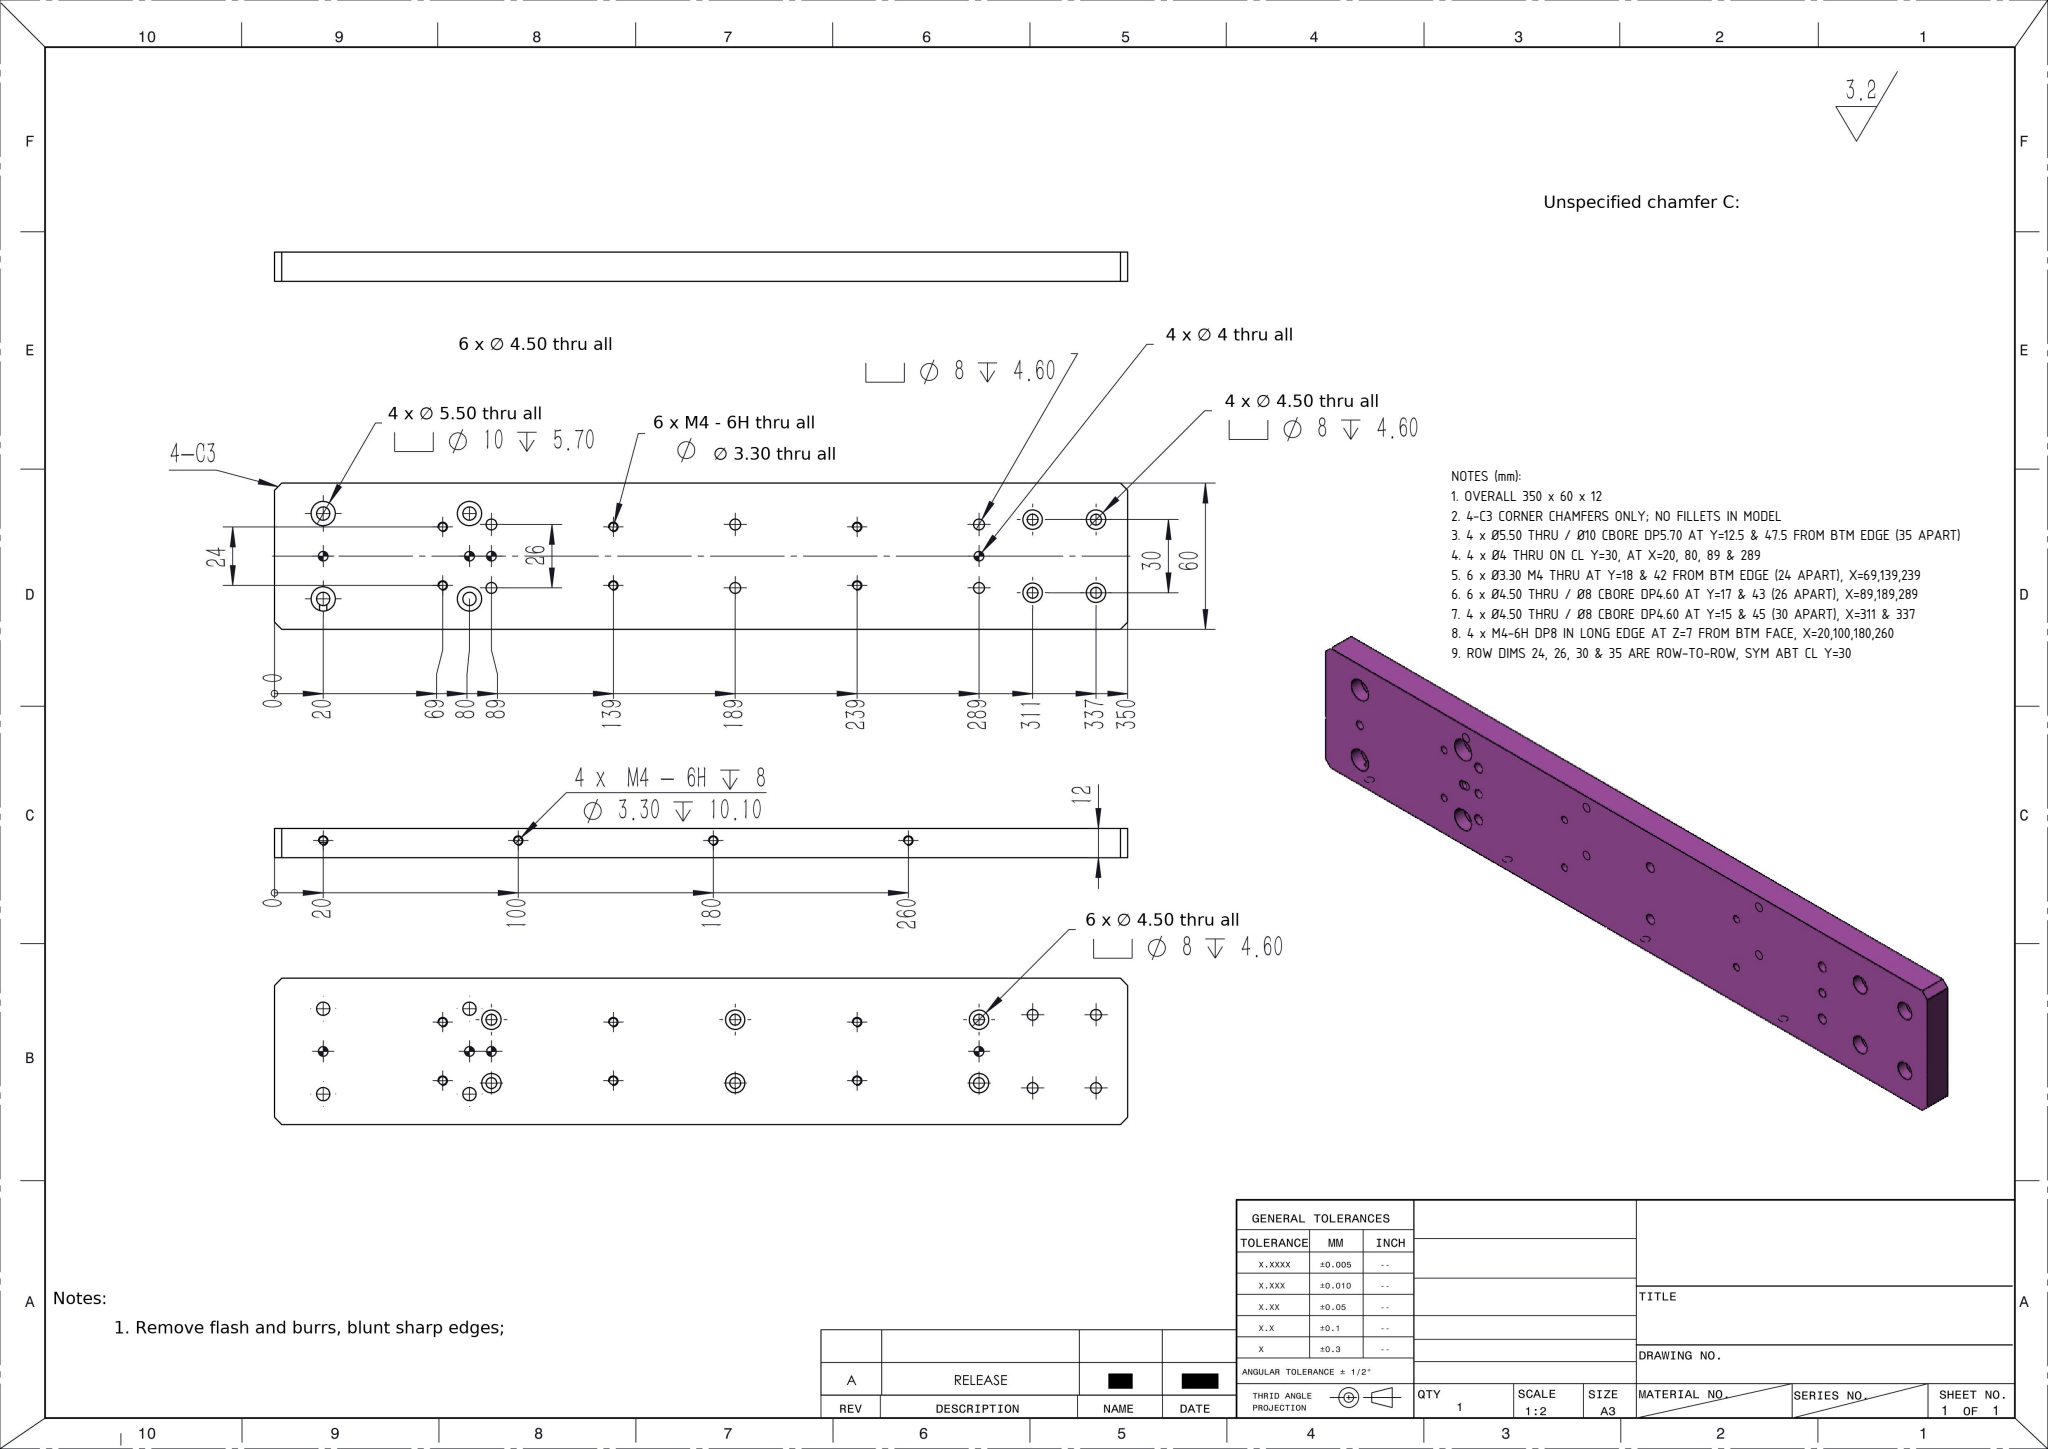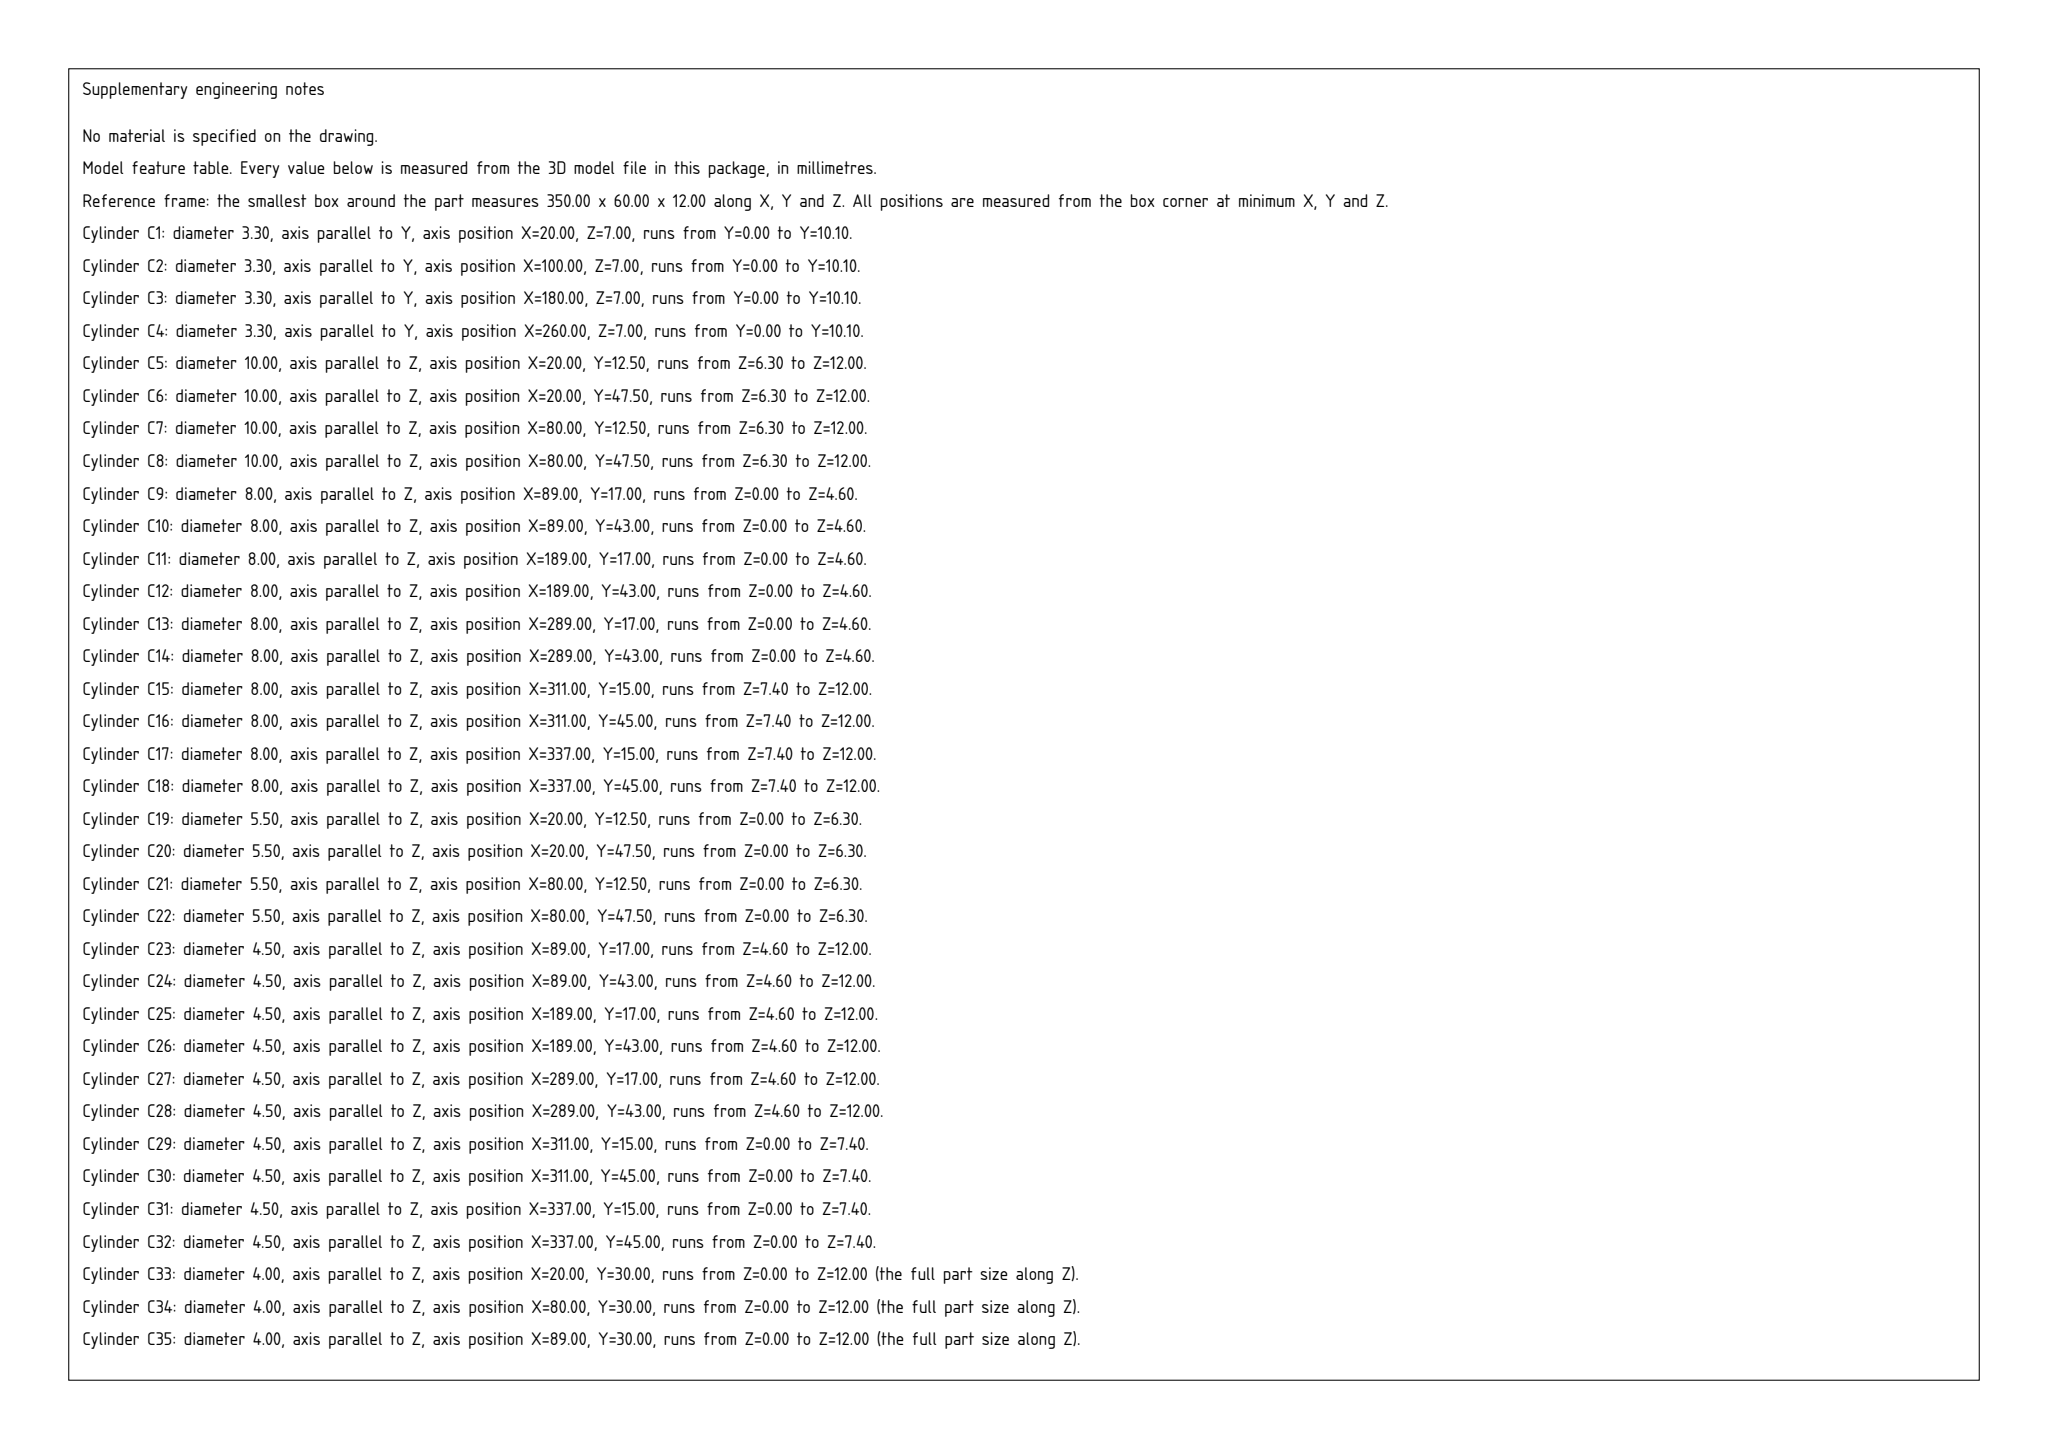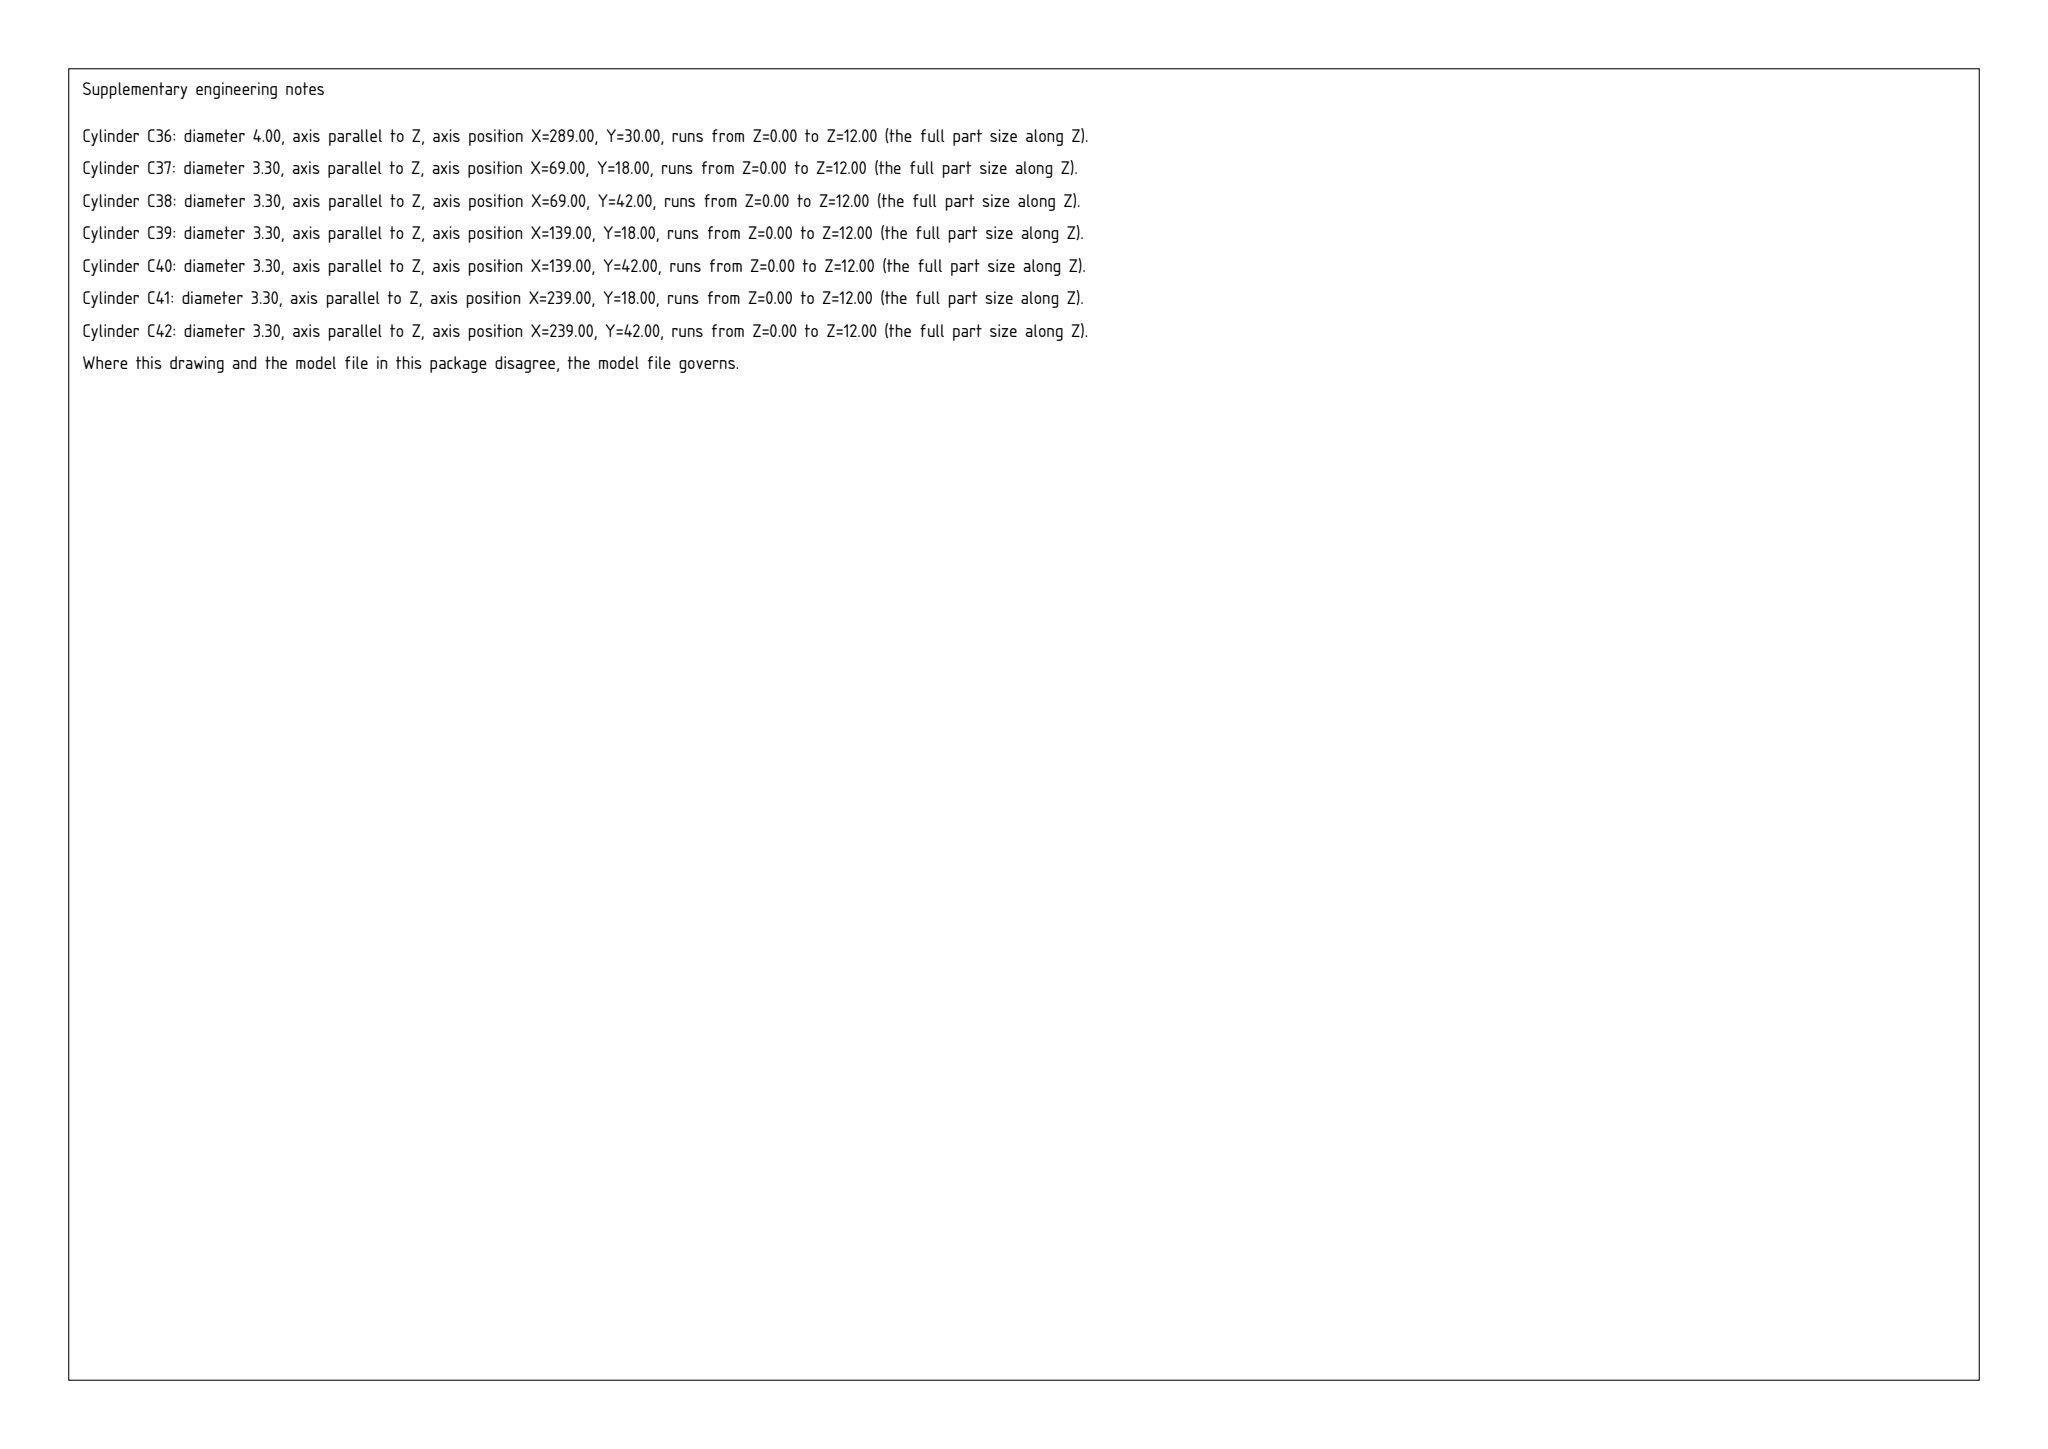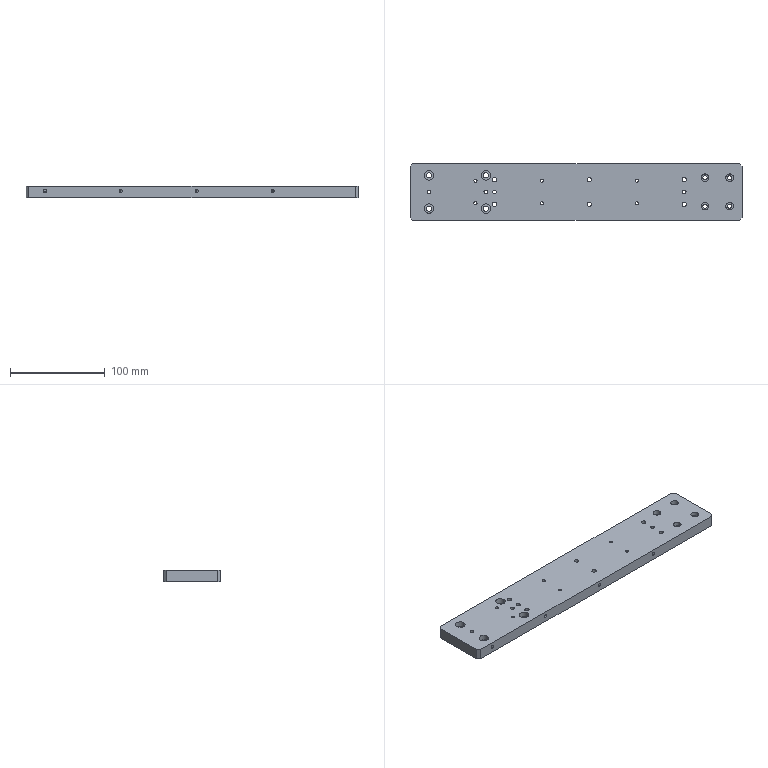Part | SolidWorks | mm | 1 solid | 116 faces | box 350 x 60 x 12 mm | volume 244349 mm3 | cylinder 84 | plane 24 | cone 8 | commonest cylinder face diameters 3.3 x20 8 x20 4.5 x20 4 x8 10 x8 5.5 x8
Drawing notes:
OVERALL 350 x 60 x 12 | from the solid: bbox_xyz 350/60/12
4-C3 CORNER CHAMFERS ONLY; NO FILLETS IN MODEL | from the solid: fillet_radii empty; only z=0 & z=12 planes plus 118 deg drill cones
4 x Ø5.50 THRU / Ø10 CBORE DP5.70 AT Y=12.5 & 47.5 FROM BTM EDGE (35 APART) | from the solid: O5.5/O10 cbores at y=12.5 and 47.5, bbox Y=60
4 x Ø4 THRU ON CL Y=30, AT X=20, 80, 89 & 289 | from the solid: O4 z-holes at [20,30],[80,30],[89,30],[289,30]
6 x Ø3.30 M4 THRU AT Y=18 & 42 FROM BTM EDGE (24 APART), X=69,139,239 | from the solid: O3.3 z-axis holes at x=69/139/239, y=18 and y=42; 42-18=24
6 x Ø4.50 THRU / Ø8 CBORE DP4.60 AT Y=17 & 43 (26 APART), X=89,189,289 | from the solid: O4.5/O8 cbores x=89,189,289 at y=17 & 43; 43-17=26
4 x Ø4.50 THRU / Ø8 CBORE DP4.60 AT Y=15 & 45 (30 APART), X=311 & 337 | from the solid: O4.5/O8 cbores x=311,337 at y=15 & 45; 45-15=30
4 x M4-6H DP8 IN LONG EDGE AT Z=7 FROM BTM FACE, X=20,100,180,260 | from the solid: O3.3 y-axis holes at z=7.0, x=20/100/180/260, len 10.1
ROW DIMS 24, 26, 30 & 35 ARE ROW-TO-ROW, SYM ABT CL Y=30 | from the solid: all hole pairs symmetric about y=30 of 60 wide plate
build123d program:
from build123d import *

# Parameters (mm, degrees)
SKETCH2_W                                         = 350
SKETCH2_H                                         = 60
BOSS_EXTRUDE1_DEPTH                               = 12
HOLE_SIZE_ACCORDING_TO_HEXAGON_SOCKET_D           = 4.5
HOLE_SIZE_ACCORDING_TO_HEXAGON_SOCKET_CBORE_D     = 8
HOLE_SIZE_ACCORDING_TO_HEXAGON_SOCKET_CBORE_DEPTH = 4.6
CHAMFER1_SIZE                                     = 3
M4_TAPPED_HOLE2_D                                 = 3.3
M4_TAPPED_HOLE2_DEPTH                             = 10.1
M4_TAPPED_HOLE2_TIP                               = 0.9914
HOLE_SIZE_ACCORDING_TO_HEXAGON_SO_2_D             = 4.5
HOLE_SIZE_ACCORDING_TO_HEXAGON_SO_2_CBORE_D       = 8
HOLE_SIZE_ACCORDING_TO_HEXAGON_SO_2_CBORE_DEPTH   = 4.6
SIZE_MM_DOWEL_PIN_HOLE0_D                         = 4
M4_TAPPED_HOLE3_D                                 = 3.3
HOLE_SIZE_ACCORDING_TO_HEXAGON_SO_3_D             = 5.5
HOLE_SIZE_ACCORDING_TO_HEXAGON_SO_3_CBORE_D       = 10
HOLE_SIZE_ACCORDING_TO_HEXAGON_SO_3_CBORE_DEPTH   = 5.7
SIZE_MM_DOWEL_PIN_HOLE1_D                         = 4


with BuildPart() as part:
    # Sketch2 → Boss-Extrude1 (new body)
    with BuildSketch(Plane.XY):
        Rectangle(SKETCH2_W, SKETCH2_H)
    extrude(amount=BOSS_EXTRUDE1_DEPTH)

    # Hole Size _ according to_ Hexagon Socket (through all)
    with Locations(Plane.XY.offset(12)):
        with Locations((136, -15), (162, -15), (136, 15), (162, 15)):
            CounterBoreHole(HOLE_SIZE_ACCORDING_TO_HEXAGON_SOCKET_D / 2, HOLE_SIZE_ACCORDING_TO_HEXAGON_SOCKET_CBORE_D / 2, HOLE_SIZE_ACCORDING_TO_HEXAGON_SOCKET_CBORE_DEPTH)

    # Chamfer1
    chamfer1_edges = [part.edges().sort_by_distance(p)[0] for p in [
        (175, -30, 6),
        (-175, -30, 6),
        (-175, 30, 6),
        (175, 30, 6),
    ]]
    chamfer(chamfer1_edges, length=CHAMFER1_SIZE)

    # M4 Tapped Hole2
    with Locations(Plane(origin=(0, -30, 0), x_dir=(-1, 0, 0), z_dir=(0, -1, 0))):
        with Locations((155, -7), (75, -7), (-5, -7), (-85, -7)):
            Hole(M4_TAPPED_HOLE2_D / 2, depth=M4_TAPPED_HOLE2_DEPTH)
            with Locations((0, 0, -(M4_TAPPED_HOLE2_DEPTH + M4_TAPPED_HOLE2_TIP / 2))):  # 118° drill point
                Cone(0, M4_TAPPED_HOLE2_D / 2, M4_TAPPED_HOLE2_TIP, mode=Mode.SUBTRACT)

    # Hole Size _ according to_ Hexagon So 2 (through all)
    with Locations(Plane(origin=(0, 0, 0), x_dir=(-1, 0, 0), z_dir=(0, 0, -1))):
        with Locations((-114, 13), (-114, -13), (-14, 13), (-14, -13), (86, 13), (86, -13)):
            CounterBoreHole(HOLE_SIZE_ACCORDING_TO_HEXAGON_SO_2_D / 2, HOLE_SIZE_ACCORDING_TO_HEXAGON_SO_2_CBORE_D / 2, HOLE_SIZE_ACCORDING_TO_HEXAGON_SO_2_CBORE_DEPTH)

    # Size mm Dowel Pin Hole0 (through all)
    with Locations(Plane(origin=(0, 0, 0), x_dir=(-1, 0, 0), z_dir=(0, 0, -1))):
        with Locations((-114, 0), (86, 0)):
            Hole(SIZE_MM_DOWEL_PIN_HOLE0_D / 2)

    # M4 Tapped Hole3 (through all)
    with Locations(Plane(origin=(0, 0, 0), x_dir=(-1, 0, 0), z_dir=(0, 0, -1))):
        with Locations((-64, 12), (-64, -12), (36, 12), (36, -12), (106, 12), (106, -12)):
            Hole(M4_TAPPED_HOLE3_D / 2)

    # Hole Size _ according to_ Hexagon So 3 (through all)
    with Locations(Plane.XY.offset(12)):
        with Locations((-155, 17.5), (-155, -17.5), (-95, 17.5), (-95, -17.5)):
            CounterBoreHole(HOLE_SIZE_ACCORDING_TO_HEXAGON_SO_3_D / 2, HOLE_SIZE_ACCORDING_TO_HEXAGON_SO_3_CBORE_D / 2, HOLE_SIZE_ACCORDING_TO_HEXAGON_SO_3_CBORE_DEPTH)

    # Size mm Dowel Pin Hole1 (through all)
    with Locations(Plane.XY.offset(12)):
        with Locations((-155, 0), (-95, 0)):
            Hole(SIZE_MM_DOWEL_PIN_HOLE1_D / 2)


solid = part.part